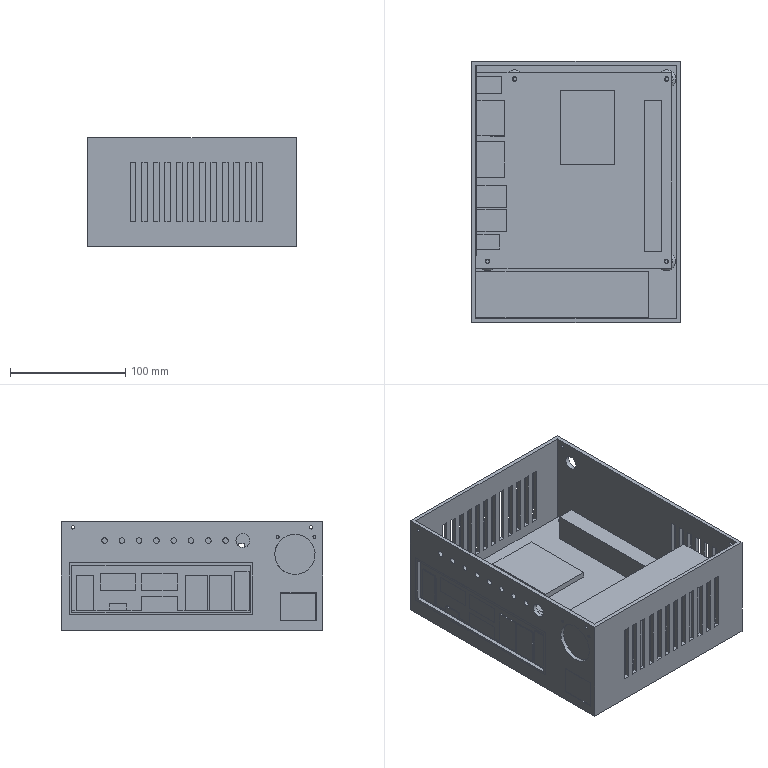Assembly | NX | mm | 12 component files | 12 solids | 422 faces | box 180.76 x 226.5 x 94.5 mm | volume 1028067 mm3 | plane 377 | cylinder 41 | cone 4 | commonest cylinder face diameters 3 x20 4.85 x8 2.61 x6 3.8 x4 12 x2 35 x1
Bill of materials:
unnamed part 1 | 4 |  | Hexagonal prism body with a round axial bore at one end and a smaller, coaxial solid cylindrical stud coming out of the other end. It looks like a male-female hex standoff.
unnamed part 2 | 4 |  | Short hexagonal prism with a central round through-hole. It looks like a plain hex nut.
unnamed part 3 | 1 |  | Solid rectangular block with a small rectangular tab sticking out from one end face, below the face's midpoint.
unnamed part 4 | 1 |  | Thin square plate with four small corner holes. Several rectangular blocks of different heights sit side by side along one edge, a long low block runs along an adjacent edge, a thin raised rectangular pad is in the interior, and a block sticks out from the underside. It looks like a simplified circuit board with block-shaped components.
unnamed part 5 | 1 |  | Thin flat rectangular plate with a short bent flange or lip along one long edge. It has a pattern of rectangular cutouts in various sizes, some split into stacked openings and one with a small notch.
unnamed part 6 | 1 |  | Open-top rectangular thin-walled box or tray. It has rows of vertical vent slots in the side walls, a large rectangular opening and a row of small holes in one long wall, a few larger round holes near the wall ends, small holes near the top corners, and four round bosses with center holes on the floor.
Mates:
1. distance | power_supply 1 face | WAIKE 1 face
2. touch align | main_board 1 face | WAIKE 1 face
3. touch align | M3_standoff 2 face | main_board 1 face
4. touch align | M3_standoff 1 face | main_board 1 face
5. touch align | M3_standoff 4 face | main_board 1 face
6. touch align | M3_standoff 3 face | main_board 1 face
7. touch align | nut 1 face | M3_standoff 2 face
8. touch align | nut 3 face | M3_standoff 1 face
9. touch align | nut 2 face | M3_standoff 4 face
10. touch align | nut 4 face | M3_standoff 3 face
11. touch align | nut 1 face | WAIKE 1 face
12. touch align | nut 3 face | WAIKE 1 face
13. touch align | nut 2 face | WAIKE 1 face
14. touch align | nut 4 face | WAIKE 1 face
15. touch align | M3_standoff 2 face | WAIKE 1 face
16. touch align | power_supply 1 face | WAIKE 1 face